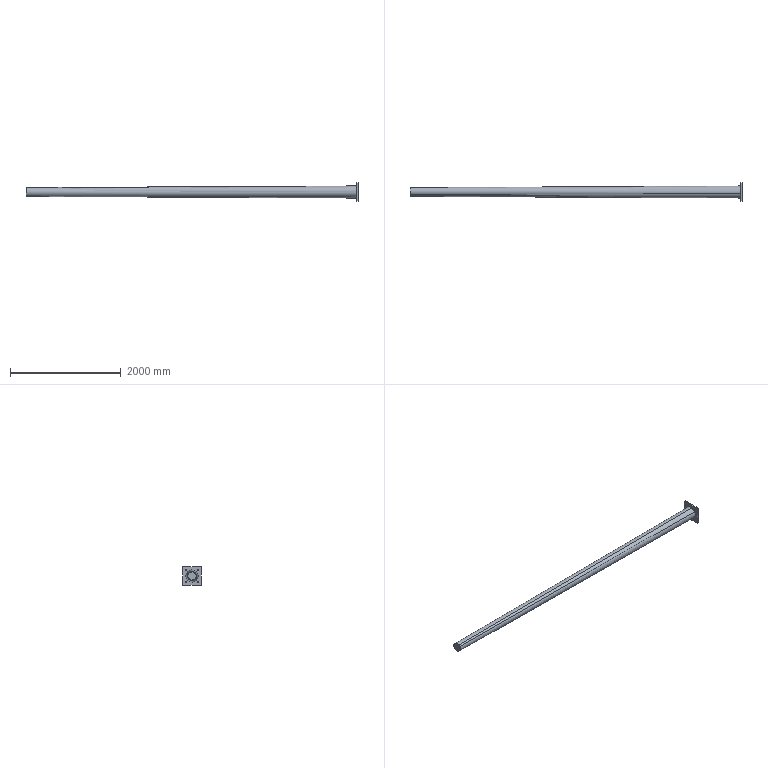Component | SolidWorks | Cantilever-1 | 1 solid | 20 faces | box 6000 x 330 x 330 mm | volume 23316974 mm3 | cylinder 8 | plane 8 | spline 2 | cone 2 | commonest cylinder face diameters 16 x8
STEP:
#1=COLOUR_RGB('',0.7922,0.8196,0.9333);
#2=FILL_AREA_STYLE_COLOUR('',#1);
#3=FILL_AREA_STYLE('',(#2));
#4=SURFACE_STYLE_FILL_AREA(#3);
#5=SURFACE_SIDE_STYLE('',(#4));
#6=SURFACE_STYLE_USAGE(.BOTH.,#5);
#7=PRESENTATION_STYLE_ASSIGNMENT((#6));
#8=CARTESIAN_POINT('',(-8.524,280.032,-4.345));
#9=VERTEX_POINT('',#8);
#10=CARTESIAN_POINT('',(-8.524,279.501,-4.007));
#11=VERTEX_POINT('',#10);
#12=CARTESIAN_POINT('',(-8.524,279.766,-4.176));
#13=DIRECTION('',(-1.,-0.,-0.));
#14=DIRECTION('',(0.,0.5373,0.8434));
#15=AXIS2_PLACEMENT_3D('',#12,#13,#14);
#16=CIRCLE('',#15,0.315);
#17=EDGE_CURVE('',#9,#11,#16,.T.);
#18=ORIENTED_EDGE('',*,*,#17,.F.);
#19=CARTESIAN_POINT('',(-9.311,280.032,-4.345));
#20=VERTEX_POINT('',#19);
#21=CARTESIAN_POINT('',(-8.524,280.032,-4.345));
#22=DIRECTION('',(-1.,-0.,-0.));
#23=VECTOR('',#22,39.37);
#24=LINE('',#21,#23);
#25=EDGE_CURVE('',#9,#20,#24,.T.);
#26=ORIENTED_EDGE('',*,*,#25,.T.);
#27=CARTESIAN_POINT('',(-9.311,279.501,-4.007));
#28=VERTEX_POINT('',#27);
#29=CARTESIAN_POINT('',(-9.311,279.766,-4.176));
#30=DIRECTION('',(-1.,-0.,-0.));
#31=DIRECTION('',(0.,0.5373,0.8434));
#32=AXIS2_PLACEMENT_3D('',#29,#30,#31);
#33=CIRCLE('',#32,0.315);
#34=EDGE_CURVE('',#20,#28,#33,.T.);
#35=ORIENTED_EDGE('',*,*,#34,.T.);
#36=CARTESIAN_POINT('',(-8.524,279.501,-4.007));
#37=DIRECTION('',(-1.,-0.,-0.));
#38=VECTOR('',#37,39.37);
#39=LINE('',#36,#38);
#40=EDGE_CURVE('',#11,#28,#39,.T.);
#41=ORIENTED_EDGE('',*,*,#40,.F.);
#42=EDGE_LOOP('',(#18,#26,#35,#41));
#43=FACE_OUTER_BOUND('',#42,.T.);
#44=CARTESIAN_POINT('',(-8.524,279.766,-4.176));
#45=DIRECTION('',(-1.,-0.,-0.));
#46=DIRECTION('',(0.,-0.8434,0.5373));
#47=AXIS2_PLACEMENT_3D('',#44,#45,#46);
#48=CYLINDRICAL_SURFACE('',#47,0.315);
#49=ADVANCED_FACE('',(#43),#48,.F.);
#50=CARTESIAN_POINT('',(-8.524,271.68,-4.345));
#51=VERTEX_POINT('',#50);
#52=CARTESIAN_POINT('',(-8.524,271.149,-4.007));
#53=VERTEX_POINT('',#52);
#54=CARTESIAN_POINT('',(-8.524,271.415,-4.176));
#55=DIRECTION('',(-1.,-0.,-0.));
#56=DIRECTION('',(0.,0.8434,-0.5373));
#57=AXIS2_PLACEMENT_3D('',#54,#55,#56);
#58=CIRCLE('',#57,0.315);
#59=EDGE_CURVE('',#51,#53,#58,.T.);
#60=ORIENTED_EDGE('',*,*,#59,.F.);
#61=CARTESIAN_POINT('',(-9.311,271.68,-4.345));
#62=VERTEX_POINT('',#61);
#63=CARTESIAN_POINT('',(-8.524,271.68,-4.345));
#64=DIRECTION('',(-1.,-0.,-0.));
#65=VECTOR('',#64,39.37);
#66=LINE('',#63,#65);
#67=EDGE_CURVE('',#51,#62,#66,.T.);
#68=ORIENTED_EDGE('',*,*,#67,.T.);
#69=CARTESIAN_POINT('',(-9.311,271.149,-4.007));
#70=VERTEX_POINT('',#69);
#71=CARTESIAN_POINT('',(-9.311,271.415,-4.176));
#72=DIRECTION('',(-1.,-0.,-0.));
#73=DIRECTION('',(0.,0.8434,-0.5373));
#74=AXIS2_PLACEMENT_3D('',#71,#72,#73);
#75=CIRCLE('',#74,0.315);
#76=EDGE_CURVE('',#62,#70,#75,.T.);
#77=ORIENTED_EDGE('',*,*,#76,.T.);
#78=CARTESIAN_POINT('',(-8.524,271.149,-4.007));
#79=DIRECTION('',(-1.,-0.,-0.));
#80=VECTOR('',#79,39.37);
#81=LINE('',#78,#80);
#82=EDGE_CURVE('',#53,#70,#81,.T.);
#83=ORIENTED_EDGE('',*,*,#82,.F.);
#84=EDGE_LOOP('',(#60,#68,#77,#83));
#85=FACE_OUTER_BOUND('',#84,.T.);
#86=CARTESIAN_POINT('',(-8.524,271.415,-4.176));
#87=DIRECTION('',(-1.,-0.,-0.));
#88=DIRECTION('',(0.,-0.8434,0.5373));
#89=AXIS2_PLACEMENT_3D('',#86,#87,#88);
#90=CYLINDRICAL_SURFACE('',#89,0.315);
#91=ADVANCED_FACE('',(#85),#90,.F.);
#92=CARTESIAN_POINT('',(-8.524,271.68,4.007));
#93=VERTEX_POINT('',#92);
#94=CARTESIAN_POINT('',(-8.524,271.149,4.345));
#95=VERTEX_POINT('',#94);
#96=CARTESIAN_POINT('',(-8.524,271.415,4.176));
#97=DIRECTION('',(-1.,-0.,-0.));
#98=DIRECTION('',(0.,-0.5373,-0.8434));
#99=AXIS2_PLACEMENT_3D('',#96,#97,#98);
#100=CIRCLE('',#99,0.315);
#101=EDGE_CURVE('',#93,#95,#100,.T.);
#102=ORIENTED_EDGE('',*,*,#101,.F.);
#103=CARTESIAN_POINT('',(-9.311,271.68,4.007));
#104=VERTEX_POINT('',#103);
#105=CARTESIAN_POINT('',(-8.524,271.68,4.007));
#106=DIRECTION('',(-1.,-0.,-0.));
#107=VECTOR('',#106,39.37);
#108=LINE('',#105,#107);
#109=EDGE_CURVE('',#93,#104,#108,.T.);
#110=ORIENTED_EDGE('',*,*,#109,.T.);
#111=CARTESIAN_POINT('',(-9.311,271.149,4.345));
#112=VERTEX_POINT('',#111);
#113=CARTESIAN_POINT('',(-9.311,271.415,4.176));
#114=DIRECTION('',(-1.,-0.,-0.));
#115=DIRECTION('',(0.,-0.5373,-0.8434));
#116=AXIS2_PLACEMENT_3D('',#113,#114,#115);
#117=CIRCLE('',#116,0.315);
#118=EDGE_CURVE('',#104,#112,#117,.T.);
#119=ORIENTED_EDGE('',*,*,#118,.T.);
#120=CARTESIAN_POINT('',(-8.524,271.149,4.345));
#121=DIRECTION('',(-1.,-0.,-0.));
#122=VECTOR('',#121,39.37);
#123=LINE('',#120,#122);
#124=EDGE_CURVE('',#95,#112,#123,.T.);
#125=ORIENTED_EDGE('',*,*,#124,.F.);
#126=EDGE_LOOP('',(#102,#110,#119,#125));
#127=FACE_OUTER_BOUND('',#126,.T.);
#128=CARTESIAN_POINT('',(-8.524,271.415,4.176));
#129=DIRECTION('',(-1.,-0.,-0.));
#130=DIRECTION('',(0.,-0.8434,0.5373));
#131=AXIS2_PLACEMENT_3D('',#128,#129,#130);
#132=CYLINDRICAL_SURFACE('',#131,0.315);
#133=ADVANCED_FACE('',(#127),#132,.F.);
#134=CARTESIAN_POINT('',(-8.524,280.032,4.007));
#135=VERTEX_POINT('',#134);
#136=CARTESIAN_POINT('',(-8.524,279.501,4.345));
#137=VERTEX_POINT('',#136);
#138=CARTESIAN_POINT('',(-8.524,279.766,4.176));
#139=DIRECTION('',(-1.,-0.,-0.));
#140=DIRECTION('',(0.,-0.8434,0.5373));
#141=AXIS2_PLACEMENT_3D('',#138,#139,#140);
#142=CIRCLE('',#141,0.315);
#143=EDGE_CURVE('',#135,#137,#142,.T.);
#144=ORIENTED_EDGE('',*,*,#143,.F.);
#145=CARTESIAN_POINT('',(-9.311,280.032,4.007));
#146=VERTEX_POINT('',#145);
#147=CARTESIAN_POINT('',(-8.524,280.032,4.007));
#148=DIRECTION('',(-1.,-0.,-0.));
#149=VECTOR('',#148,39.37);
#150=LINE('',#147,#149);
#151=EDGE_CURVE('',#135,#146,#150,.T.);
#152=ORIENTED_EDGE('',*,*,#151,.T.);
#153=CARTESIAN_POINT('',(-9.311,279.501,4.345));
#154=VERTEX_POINT('',#153);
#155=CARTESIAN_POINT('',(-9.311,279.766,4.176));
#156=DIRECTION('',(-1.,-0.,-0.));
#157=DIRECTION('',(0.,-0.8434,0.5373));
#158=AXIS2_PLACEMENT_3D('',#155,#156,#157);
#159=CIRCLE('',#158,0.315);
#160=EDGE_CURVE('',#146,#154,#159,.T.);
#161=ORIENTED_EDGE('',*,*,#160,.T.);
#162=CARTESIAN_POINT('',(-8.524,279.501,4.345));
#163=DIRECTION('',(-1.,-0.,-0.));
#164=VECTOR('',#163,39.37);
#165=LINE('',#162,#164);
#166=EDGE_CURVE('',#137,#154,#165,.T.);
#167=ORIENTED_EDGE('',*,*,#166,.F.);
#168=EDGE_LOOP('',(#144,#152,#161,#167));
#169=FACE_OUTER_BOUND('',#168,.T.);
#170=CARTESIAN_POINT('',(-8.524,279.766,4.176));
#171=DIRECTION('',(-1.,-0.,-0.));
#172=DIRECTION('',(0.,-0.8434,0.5373));
#173=AXIS2_PLACEMENT_3D('',#170,#171,#172);
#174=CYLINDRICAL_SURFACE('',#173,0.315);
#175=ADVANCED_FACE('',(#169),#174,.F.);
#176=CARTESIAN_POINT('',(-244.744,277.198,-2.686));
#177=VERTEX_POINT('',#176);
#178=CARTESIAN_POINT('',(-244.744,273.983,2.686));
#179=VERTEX_POINT('',#178);
#180=CARTESIAN_POINT('',(-244.744,275.591,0.));
#181=DIRECTION('',(-1.,-0.,-0.));
#182=DIRECTION('',(0.,-0.8434,0.5373));
#183=AXIS2_PLACEMENT_3D('',#180,#181,#182);
#184=CIRCLE('',#183,3.13);
#185=EDGE_CURVE('',#177,#179,#184,.T.);
#186=ORIENTED_EDGE('',*,*,#185,.F.);
#187=CARTESIAN_POINT('',(-9.311,276.61,-4.184));
#188=VERTEX_POINT('',#187);
#189=CARTESIAN_POINT('',(-244.744,277.198,-2.686));
#190=CARTESIAN_POINT('',(-9.311,276.61,-4.184));
#191=B_SPLINE_CURVE_WITH_KNOTS('',1,(#189,#190),.UNSPECIFIED.,.F.,.F.,(2,2),(0.,0.9967),.UNSPECIFIED.);
#192=EDGE_CURVE('',#177,#188,#191,.T.);
#193=ORIENTED_EDGE('',*,*,#192,.T.);
#194=CARTESIAN_POINT('',(-9.311,274.571,4.184));
#195=VERTEX_POINT('',#194);
#196=CARTESIAN_POINT('',(-9.311,275.591,0.));
#197=DIRECTION('',(-1.,-0.,-0.));
#198=DIRECTION('',(0.,0.8434,-0.5373));
#199=AXIS2_PLACEMENT_3D('',#196,#197,#198);
#200=CIRCLE('',#199,4.307);
#201=EDGE_CURVE('',#188,#195,#200,.T.);
#202=ORIENTED_EDGE('',*,*,#201,.T.);
#203=CARTESIAN_POINT('',(-244.744,273.983,2.686));
#204=CARTESIAN_POINT('',(-9.311,274.571,4.184));
#205=B_SPLINE_CURVE_WITH_KNOTS('',1,(#203,#204),.UNSPECIFIED.,.F.,.F.,(2,2),(0.,0.9967),.UNSPECIFIED.);
#206=EDGE_CURVE('',#179,#195,#205,.T.);
#207=ORIENTED_EDGE('',*,*,#206,.F.);
#208=EDGE_LOOP('',(#186,#193,#202,#207));
#209=FACE_OUTER_BOUND('',#208,.T.);
#210=CARTESIAN_POINT('',(-244.744,273.983,2.686));
#211=CARTESIAN_POINT('',(-8.524,274.573,4.189));
#212=CARTESIAN_POINT('',(-244.744,268.612,-0.5283));
#213=CARTESIAN_POINT('',(-8.524,266.195,2.155));
#214=CARTESIAN_POINT('',(-244.744,271.826,-5.9));
#215=CARTESIAN_POINT('',(-8.524,268.229,-6.224));
#216=CARTESIAN_POINT('',(-244.744,277.198,-2.686));
#217=CARTESIAN_POINT('',(-8.524,276.608,-4.189));
#218=CARTESIAN_POINT('',(-244.744,282.569,0.5283));
#219=CARTESIAN_POINT('',(-8.524,284.986,-2.155));
#220=CARTESIAN_POINT('',(-244.744,279.355,5.9));
#221=CARTESIAN_POINT('',(-8.524,282.952,6.224));
#222=CARTESIAN_POINT('',(-244.744,273.983,2.686));
#223=CARTESIAN_POINT('',(-8.524,274.573,4.189));
#224=(BOUNDED_SURFACE()B_SPLINE_SURFACE(3,1,((#210,#211),(#212,#213),(#214,#215),(#216,#217),(#218,#219),(#220,#221),(#222,#223)),.UNSPECIFIED.,.T.,.F.,.T.)B_SPLINE_SURFACE_WITH_KNOTS((4,3,4),(2,2),(0.,0.5,1.),(0.,1.),.UNSPECIFIED.)GEOMETRIC_REPRESENTATION_ITEM()RATIONAL_B_SPLINE_SURFACE(((1.,1.),(0.3333,0.3333),(0.3333,0.3333),(1.,1.),(0.3333,0.3333),(0.3333,0.3333),(1.,1.)))REPRESENTATION_ITEM('')SURFACE());
#225=ADVANCED_FACE('',(#209),#224,.T.);
#226=CARTESIAN_POINT('',(-244.35,273.149,1.556));
#227=VERTEX_POINT('',#226);
#228=CARTESIAN_POINT('',(-244.35,278.033,-1.556));
#229=VERTEX_POINT('',#228);
#230=CARTESIAN_POINT('',(-244.35,275.591,0.));
#231=DIRECTION('',(1.,0.,0.));
#232=DIRECTION('',(0.,-0.8434,0.5373));
#233=AXIS2_PLACEMENT_3D('',#230,#231,#232);
#234=CIRCLE('',#233,2.896);
#235=EDGE_CURVE('',#227,#229,#234,.T.);
#236=ORIENTED_EDGE('',*,*,#235,.F.);
#237=CARTESIAN_POINT('',(-8.524,272.22,2.147));
#238=VERTEX_POINT('',#237);
#239=CARTESIAN_POINT('',(-244.744,273.15,1.555));
#240=DIRECTION('',(1.,-0.003936,0.002507));
#241=VECTOR('',#240,39.37);
#242=LINE('',#239,#241);
#243=EDGE_CURVE('',#227,#238,#242,.T.);
#244=ORIENTED_EDGE('',*,*,#243,.T.);
#245=CARTESIAN_POINT('',(-8.524,278.961,-2.147));
#246=VERTEX_POINT('',#245);
#247=CARTESIAN_POINT('',(-8.524,275.591,0.));
#248=DIRECTION('',(-1.,-0.,-0.));
#249=DIRECTION('',(0.,-0.8434,0.5373));
#250=AXIS2_PLACEMENT_3D('',#247,#248,#249);
#251=CIRCLE('',#250,3.996);
#252=EDGE_CURVE('',#246,#238,#251,.T.);
#253=ORIENTED_EDGE('',*,*,#252,.F.);
#254=CARTESIAN_POINT('',(-244.744,278.031,-1.555));
#255=DIRECTION('',(1.,0.003936,-0.002507));
#256=VECTOR('',#255,39.37);
#257=LINE('',#254,#256);
#258=EDGE_CURVE('',#229,#246,#257,.T.);
#259=ORIENTED_EDGE('',*,*,#258,.F.);
#260=EDGE_LOOP('',(#236,#244,#253,#259));
#261=FACE_OUTER_BOUND('',#260,.T.);
#262=CARTESIAN_POINT('',(-244.744,275.591,0.));
#263=DIRECTION('',(1.,0.,0.));
#264=DIRECTION('',(0.,0.8434,-0.5373));
#265=AXIS2_PLACEMENT_3D('',#262,#263,#264);
#266=CONICAL_SURFACE('',#265,2.894,0.004667);
#267=ADVANCED_FACE('',(#261),#266,.F.);
#268=ORIENTED_EDGE('',*,*,#243,.F.);
#269=CARTESIAN_POINT('',(-244.35,275.591,0.));
#270=DIRECTION('',(1.,0.,0.));
#271=DIRECTION('',(0.,-0.8434,0.5373));
#272=AXIS2_PLACEMENT_3D('',#269,#270,#271);
#273=CIRCLE('',#272,2.896);
#274=EDGE_CURVE('',#229,#227,#273,.T.);
#275=ORIENTED_EDGE('',*,*,#274,.F.);
#276=ORIENTED_EDGE('',*,*,#258,.T.);
#277=CARTESIAN_POINT('',(-8.524,275.591,0.));
#278=DIRECTION('',(-1.,-0.,-0.));
#279=DIRECTION('',(0.,-0.8434,0.5373));
#280=AXIS2_PLACEMENT_3D('',#277,#278,#279);
#281=CIRCLE('',#280,3.996);
#282=EDGE_CURVE('',#238,#246,#281,.T.);
#283=ORIENTED_EDGE('',*,*,#282,.F.);
#284=EDGE_LOOP('',(#268,#275,#276,#283));
#285=FACE_OUTER_BOUND('',#284,.T.);
#286=CARTESIAN_POINT('',(-244.744,275.591,0.));
#287=DIRECTION('',(1.,0.,0.));
#288=DIRECTION('',(0.,0.8434,-0.5373));
#289=AXIS2_PLACEMENT_3D('',#286,#287,#288);
#290=CONICAL_SURFACE('',#289,2.894,0.004667);
#291=ADVANCED_FACE('',(#285),#290,.F.);
#292=ORIENTED_EDGE('',*,*,#192,.F.);
#293=CARTESIAN_POINT('',(-244.744,275.591,0.));
#294=DIRECTION('',(-1.,-0.,-0.));
#295=DIRECTION('',(0.,-0.8434,0.5373));
#296=AXIS2_PLACEMENT_3D('',#293,#294,#295);
#297=CIRCLE('',#296,3.13);
#298=EDGE_CURVE('',#179,#177,#297,.T.);
#299=ORIENTED_EDGE('',*,*,#298,.F.);
#300=ORIENTED_EDGE('',*,*,#206,.T.);
#301=CARTESIAN_POINT('',(-9.311,275.591,0.));
#302=DIRECTION('',(-1.,-0.,-0.));
#303=DIRECTION('',(0.,0.8434,-0.5373));
#304=AXIS2_PLACEMENT_3D('',#301,#302,#303);
#305=CIRCLE('',#304,4.307);
#306=EDGE_CURVE('',#195,#188,#305,.T.);
#307=ORIENTED_EDGE('',*,*,#306,.T.);
#308=EDGE_LOOP('',(#292,#299,#300,#307));
#309=FACE_OUTER_BOUND('',#308,.T.);
#310=CARTESIAN_POINT('',(-244.744,273.983,2.686));
#311=CARTESIAN_POINT('',(-8.524,274.573,4.189));
#312=CARTESIAN_POINT('',(-244.744,268.612,-0.5283));
#313=CARTESIAN_POINT('',(-8.524,266.195,2.155));
#314=CARTESIAN_POINT('',(-244.744,271.826,-5.9));
#315=CARTESIAN_POINT('',(-8.524,268.229,-6.224));
#316=CARTESIAN_POINT('',(-244.744,277.198,-2.686));
#317=CARTESIAN_POINT('',(-8.524,276.608,-4.189));
#318=CARTESIAN_POINT('',(-244.744,282.569,0.5283));
#319=CARTESIAN_POINT('',(-8.524,284.986,-2.155));
#320=CARTESIAN_POINT('',(-244.744,279.355,5.9));
#321=CARTESIAN_POINT('',(-8.524,282.952,6.224));
#322=CARTESIAN_POINT('',(-244.744,273.983,2.686));
#323=CARTESIAN_POINT('',(-8.524,274.573,4.189));
#324=(BOUNDED_SURFACE()B_SPLINE_SURFACE(3,1,((#310,#311),(#312,#313),(#314,#315),(#316,#317),(#318,#319),(#320,#321),(#322,#323)),.UNSPECIFIED.,.T.,.F.,.F.)B_SPLINE_SURFACE_WITH_KNOTS((4,3,4),(2,2),(0.,0.5,1.),(0.,1.),.UNSPECIFIED.)GEOMETRIC_REPRESENTATION_ITEM()RATIONAL_B_SPLINE_SURFACE(((1.,1.),(0.3333,0.3333),(0.3333,0.3333),(1.,1.),(0.3333,0.3333),(0.3333,0.3333),(1.,1.)))REPRESENTATION_ITEM('')SURFACE());
#325=ADVANCED_FACE('',(#309),#324,.T.);
#326=CARTESIAN_POINT('',(-8.524,279.766,-4.176));
#327=DIRECTION('',(-1.,-0.,-0.));
#328=DIRECTION('',(0.,0.5373,0.8434));
#329=AXIS2_PLACEMENT_3D('',#326,#327,#328);
#330=CIRCLE('',#329,0.315);
#331=EDGE_CURVE('',#11,#9,#330,.T.);
#332=ORIENTED_EDGE('',*,*,#331,.T.);
#333=ORIENTED_EDGE('',*,*,#17,.T.);
#334=EDGE_LOOP('',(#332,#333));
#335=FACE_BOUND('',#334,.T.);
#336=CARTESIAN_POINT('',(-8.524,271.415,-4.176));
#337=DIRECTION('',(-1.,-0.,-0.));
#338=DIRECTION('',(0.,0.8434,-0.5373));
#339=AXIS2_PLACEMENT_3D('',#336,#337,#338);
#340=CIRCLE('',#339,0.315);
#341=EDGE_CURVE('',#53,#51,#340,.T.);
#342=ORIENTED_EDGE('',*,*,#341,.T.);
#343=ORIENTED_EDGE('',*,*,#59,.T.);
#344=EDGE_LOOP('',(#342,#343));
#345=FACE_BOUND('',#344,.T.);
#346=CARTESIAN_POINT('',(-8.524,271.415,4.176));
#347=DIRECTION('',(-1.,-0.,-0.));
#348=DIRECTION('',(0.,-0.5373,-0.8434));
#349=AXIS2_PLACEMENT_3D('',#346,#347,#348);
#350=CIRCLE('',#349,0.315);
#351=EDGE_CURVE('',#95,#93,#350,.T.);
#352=ORIENTED_EDGE('',*,*,#351,.T.);
#353=ORIENTED_EDGE('',*,*,#101,.T.);
#354=EDGE_LOOP('',(#352,#353));
#355=FACE_BOUND('',#354,.T.);
#356=CARTESIAN_POINT('',(-8.524,279.766,4.176));
#357=DIRECTION('',(-1.,-0.,-0.));
#358=DIRECTION('',(0.,-0.8434,0.5373));
#359=AXIS2_PLACEMENT_3D('',#356,#357,#358);
#360=CIRCLE('',#359,0.315);
#361=EDGE_CURVE('',#137,#135,#360,.T.);
#362=ORIENTED_EDGE('',*,*,#361,.T.);
#363=ORIENTED_EDGE('',*,*,#143,.T.);
#364=EDGE_LOOP('',(#362,#363));
#365=FACE_BOUND('',#364,.T.);
#366=ORIENTED_EDGE('',*,*,#252,.T.);
#367=ORIENTED_EDGE('',*,*,#282,.T.);
#368=EDGE_LOOP('',(#366,#367));
#369=FACE_BOUND('',#368,.T.);
#370=CARTESIAN_POINT('',(-8.524,269.094,-6.496));
#371=VERTEX_POINT('',#370);
#372=CARTESIAN_POINT('',(-8.524,282.087,-6.496));
#373=VERTEX_POINT('',#372);
#374=CARTESIAN_POINT('',(-8.524,269.094,-6.496));
#375=DIRECTION('',(-0.,1.,0.));
#376=VECTOR('',#375,39.37);
#377=LINE('',#374,#376);
#378=EDGE_CURVE('',#371,#373,#377,.T.);
#379=ORIENTED_EDGE('',*,*,#378,.T.);
#380=CARTESIAN_POINT('',(-8.524,282.087,6.496));
#381=VERTEX_POINT('',#380);
#382=CARTESIAN_POINT('',(-8.524,282.087,-6.496));
#383=DIRECTION('',(-0.,-0.,1.));
#384=VECTOR('',#383,39.37);
#385=LINE('',#382,#384);
#386=EDGE_CURVE('',#373,#381,#385,.T.);
#387=ORIENTED_EDGE('',*,*,#386,.T.);
#388=CARTESIAN_POINT('',(-8.524,269.094,6.496));
#389=VERTEX_POINT('',#388);
#390=CARTESIAN_POINT('',(-8.524,282.087,6.496));
#391=DIRECTION('',(0.,-1.,0.));
#392=VECTOR('',#391,39.37);
#393=LINE('',#390,#392);
#394=EDGE_CURVE('',#381,#389,#393,.T.);
#395=ORIENTED_EDGE('',*,*,#394,.T.);
#396=CARTESIAN_POINT('',(-8.524,269.094,6.496));
#397=DIRECTION('',(0.,0.,-1.));
#398=VECTOR('',#397,39.37);
#399=LINE('',#396,#398);
#400=EDGE_CURVE('',#389,#371,#399,.T.);
#401=ORIENTED_EDGE('',*,*,#400,.T.);
#402=EDGE_LOOP('',(#379,#387,#395,#401));
#403=FACE_OUTER_BOUND('',#402,.T.);
#404=CARTESIAN_POINT('',(-8.524,275.591,0.));
#405=DIRECTION('',(-1.,-0.,-0.));
#406=DIRECTION('',(0.,-0.8434,0.5373));
#407=AXIS2_PLACEMENT_3D('',#404,#405,#406);
#408=PLANE('',#407);
#409=ADVANCED_FACE('',(#335,#345,#355,#365,#369,#403),#408,.F.);
#410=ORIENTED_EDGE('',*,*,#298,.T.);
#411=ORIENTED_EDGE('',*,*,#185,.T.);
#412=EDGE_LOOP('',(#410,#411));
#413=FACE_OUTER_BOUND('',#412,.T.);
#414=CARTESIAN_POINT('',(-244.744,275.591,0.));
#415=DIRECTION('',(-1.,-0.,-0.));
#416=DIRECTION('',(0.,-0.8434,0.5373));
#417=AXIS2_PLACEMENT_3D('',#414,#415,#416);
#418=PLANE('',#417);
#419=ADVANCED_FACE('',(#413),#418,.T.);
#420=ORIENTED_EDGE('',*,*,#378,.F.);
#421=CARTESIAN_POINT('',(-9.311,269.094,-6.496));
#422=VERTEX_POINT('',#421);
#423=CARTESIAN_POINT('',(-9.311,269.094,-6.496));
#424=DIRECTION('',(1.,0.,0.));
#425=VECTOR('',#424,39.37);
#426=LINE('',#423,#425);
#427=EDGE_CURVE('',#422,#371,#426,.T.);
#428=ORIENTED_EDGE('',*,*,#427,.F.);
#429=CARTESIAN_POINT('',(-9.311,282.087,-6.496));
#430=VERTEX_POINT('',#429);
#431=CARTESIAN_POINT('',(-9.311,269.094,-6.496));
#432=DIRECTION('',(-0.,1.,0.));
#433=VECTOR('',#432,39.37);
#434=LINE('',#431,#433);
#435=EDGE_CURVE('',#422,#430,#434,.T.);
#436=ORIENTED_EDGE('',*,*,#435,.T.);
#437=CARTESIAN_POINT('',(-9.311,282.087,-6.496));
#438=DIRECTION('',(1.,0.,0.));
#439=VECTOR('',#438,39.37);
#440=LINE('',#437,#439);
#441=EDGE_CURVE('',#430,#373,#440,.T.);
#442=ORIENTED_EDGE('',*,*,#441,.T.);
#443=EDGE_LOOP('',(#420,#428,#436,#442));
#444=FACE_OUTER_BOUND('',#443,.T.);
#445=CARTESIAN_POINT('',(-9.311,269.094,-6.496));
#446=DIRECTION('',(0.,0.,-1.));
#447=DIRECTION('',(0.,-1.,-0.));
#448=AXIS2_PLACEMENT_3D('',#445,#446,#447);
#449=PLANE('',#448);
#450=ADVANCED_FACE('',(#444),#449,.T.);
#451=ORIENTED_EDGE('',*,*,#400,.F.);
#452=CARTESIAN_POINT('',(-9.311,269.094,6.496));
#453=VERTEX_POINT('',#452);
#454=CARTESIAN_POINT('',(-9.311,269.094,6.496));
#455=DIRECTION('',(1.,0.,0.));
#456=VECTOR('',#455,39.37);
#457=LINE('',#454,#456);
#458=EDGE_CURVE('',#453,#389,#457,.T.);
#459=ORIENTED_EDGE('',*,*,#458,.F.);
#460=CARTESIAN_POINT('',(-9.311,269.094,6.496));
#461=DIRECTION('',(0.,0.,-1.));
#462=VECTOR('',#461,39.37);
#463=LINE('',#460,#462);
#464=EDGE_CURVE('',#453,#422,#463,.T.);
#465=ORIENTED_EDGE('',*,*,#464,.T.);
#466=ORIENTED_EDGE('',*,*,#427,.T.);
#467=EDGE_LOOP('',(#451,#459,#465,#466));
#468=FACE_OUTER_BOUND('',#467,.T.);
#469=CARTESIAN_POINT('',(-9.311,269.094,6.496));
#470=DIRECTION('',(0.,-1.,-0.));
#471=DIRECTION('',(-0.,-0.,1.));
#472=AXIS2_PLACEMENT_3D('',#469,#470,#471);
#473=PLANE('',#472);
#474=ADVANCED_FACE('',(#468),#473,.T.);
#475=ORIENTED_EDGE('',*,*,#394,.F.);
#476=CARTESIAN_POINT('',(-9.311,282.087,6.496));
#477=VERTEX_POINT('',#476);
#478=CARTESIAN_POINT('',(-9.311,282.087,6.496));
#479=DIRECTION('',(1.,0.,0.));
#480=VECTOR('',#479,39.37);
#481=LINE('',#478,#480);
#482=EDGE_CURVE('',#477,#381,#481,.T.);
#483=ORIENTED_EDGE('',*,*,#482,.F.);
#484=CARTESIAN_POINT('',(-9.311,282.087,6.496));
#485=DIRECTION('',(0.,-1.,0.));
#486=VECTOR('',#485,39.37);
#487=LINE('',#484,#486);
#488=EDGE_CURVE('',#477,#453,#487,.T.);
#489=ORIENTED_EDGE('',*,*,#488,.T.);
#490=ORIENTED_EDGE('',*,*,#458,.T.);
#491=EDGE_LOOP('',(#475,#483,#489,#490));
#492=FACE_OUTER_BOUND('',#491,.T.);
#493=CARTESIAN_POINT('',(-9.311,282.087,6.496));
#494=DIRECTION('',(-0.,0.,1.));
#495=DIRECTION('',(-0.,1.,-0.));
#496=AXIS2_PLACEMENT_3D('',#493,#494,#495);
#497=PLANE('',#496);
#498=ADVANCED_FACE('',(#492),#497,.T.);
#499=ORIENTED_EDGE('',*,*,#386,.F.);
#500=ORIENTED_EDGE('',*,*,#441,.F.);
#501=CARTESIAN_POINT('',(-9.311,282.087,-6.496));
#502=DIRECTION('',(-0.,-0.,1.));
#503=VECTOR('',#502,39.37);
#504=LINE('',#501,#503);
#505=EDGE_CURVE('',#430,#477,#504,.T.);
#506=ORIENTED_EDGE('',*,*,#505,.T.);
#507=ORIENTED_EDGE('',*,*,#482,.T.);
#508=EDGE_LOOP('',(#499,#500,#506,#507));
#509=FACE_OUTER_BOUND('',#508,.T.);
#510=CARTESIAN_POINT('',(-9.311,282.087,-6.496));
#511=DIRECTION('',(-0.,1.,0.));
#512=DIRECTION('',(0.,0.,-1.));
#513=AXIS2_PLACEMENT_3D('',#510,#511,#512);
#514=PLANE('',#513);
#515=ADVANCED_FACE('',(#509),#514,.T.);
#516=CARTESIAN_POINT('',(-9.311,279.766,-4.176));
#517=DIRECTION('',(-1.,-0.,-0.));
#518=DIRECTION('',(0.,0.5373,0.8434));
#519=AXIS2_PLACEMENT_3D('',#516,#517,#518);
#520=CIRCLE('',#519,0.315);
#521=EDGE_CURVE('',#28,#20,#520,.T.);
#522=ORIENTED_EDGE('',*,*,#521,.F.);
#523=ORIENTED_EDGE('',*,*,#34,.F.);
#524=EDGE_LOOP('',(#522,#523));
#525=FACE_BOUND('',#524,.T.);
#526=CARTESIAN_POINT('',(-9.311,271.415,-4.176));
#527=DIRECTION('',(-1.,-0.,-0.));
#528=DIRECTION('',(0.,0.8434,-0.5373));
#529=AXIS2_PLACEMENT_3D('',#526,#527,#528);
#530=CIRCLE('',#529,0.315);
#531=EDGE_CURVE('',#70,#62,#530,.T.);
#532=ORIENTED_EDGE('',*,*,#531,.F.);
#533=ORIENTED_EDGE('',*,*,#76,.F.);
#534=EDGE_LOOP('',(#532,#533));
#535=FACE_BOUND('',#534,.T.);
#536=CARTESIAN_POINT('',(-9.311,271.415,4.176));
#537=DIRECTION('',(-1.,-0.,-0.));
#538=DIRECTION('',(0.,-0.5373,-0.8434));
#539=AXIS2_PLACEMENT_3D('',#536,#537,#538);
#540=CIRCLE('',#539,0.315);
#541=EDGE_CURVE('',#112,#104,#540,.T.);
#542=ORIENTED_EDGE('',*,*,#541,.F.);
#543=ORIENTED_EDGE('',*,*,#118,.F.);
#544=EDGE_LOOP('',(#542,#543));
#545=FACE_BOUND('',#544,.T.);
#546=CARTESIAN_POINT('',(-9.311,279.766,4.176));
#547=DIRECTION('',(-1.,-0.,-0.));
#548=DIRECTION('',(0.,-0.8434,0.5373));
#549=AXIS2_PLACEMENT_3D('',#546,#547,#548);
#550=CIRCLE('',#549,0.315);
#551=EDGE_CURVE('',#154,#146,#550,.T.);
#552=ORIENTED_EDGE('',*,*,#551,.F.);
#553=ORIENTED_EDGE('',*,*,#160,.F.);
#554=EDGE_LOOP('',(#552,#553));
#555=FACE_BOUND('',#554,.T.);
#556=ORIENTED_EDGE('',*,*,#306,.F.);
#557=ORIENTED_EDGE('',*,*,#201,.F.);
#558=EDGE_LOOP('',(#556,#557));
#559=FACE_BOUND('',#558,.T.);
#560=ORIENTED_EDGE('',*,*,#435,.F.);
#561=ORIENTED_EDGE('',*,*,#464,.F.);
#562=ORIENTED_EDGE('',*,*,#488,.F.);
#563=ORIENTED_EDGE('',*,*,#505,.F.);
#564=EDGE_LOOP('',(#560,#561,#562,#563));
#565=FACE_OUTER_BOUND('',#564,.T.);
#566=CARTESIAN_POINT('',(-9.311,108.152,-262.807));
#567=DIRECTION('',(1.,0.,0.));
#568=DIRECTION('',(-0.,0.8434,-0.5373));
#569=AXIS2_PLACEMENT_3D('',#566,#567,#568);
#570=PLANE('',#569);
#571=ADVANCED_FACE('',(#525,#535,#545,#555,#559,#565),#570,.F.);
#572=ORIENTED_EDGE('',*,*,#151,.F.);
#573=ORIENTED_EDGE('',*,*,#361,.F.);
#574=ORIENTED_EDGE('',*,*,#166,.T.);
#575=ORIENTED_EDGE('',*,*,#551,.T.);
#576=EDGE_LOOP('',(#572,#573,#574,#575));
#577=FACE_OUTER_BOUND('',#576,.T.);
#578=CARTESIAN_POINT('',(-8.524,279.766,4.176));
#579=DIRECTION('',(-1.,-0.,-0.));
#580=DIRECTION('',(0.,-0.8434,0.5373));
#581=AXIS2_PLACEMENT_3D('',#578,#579,#580);
#582=CYLINDRICAL_SURFACE('',#581,0.315);
#583=ADVANCED_FACE('',(#577),#582,.F.);
#584=ORIENTED_EDGE('',*,*,#109,.F.);
#585=ORIENTED_EDGE('',*,*,#351,.F.);
#586=ORIENTED_EDGE('',*,*,#124,.T.);
#587=ORIENTED_EDGE('',*,*,#541,.T.);
#588=EDGE_LOOP('',(#584,#585,#586,#587));
#589=FACE_OUTER_BOUND('',#588,.T.);
#590=CARTESIAN_POINT('',(-8.524,271.415,4.176));
#591=DIRECTION('',(-1.,-0.,-0.));
#592=DIRECTION('',(0.,-0.8434,0.5373));
#593=AXIS2_PLACEMENT_3D('',#590,#591,#592);
#594=CYLINDRICAL_SURFACE('',#593,0.315);
#595=ADVANCED_FACE('',(#589),#594,.F.);
#596=ORIENTED_EDGE('',*,*,#67,.F.);
#597=ORIENTED_EDGE('',*,*,#341,.F.);
#598=ORIENTED_EDGE('',*,*,#82,.T.);
#599=ORIENTED_EDGE('',*,*,#531,.T.);
#600=EDGE_LOOP('',(#596,#597,#598,#599));
#601=FACE_OUTER_BOUND('',#600,.T.);
#602=CARTESIAN_POINT('',(-8.524,271.415,-4.176));
#603=DIRECTION('',(-1.,-0.,-0.));
#604=DIRECTION('',(0.,-0.8434,0.5373));
#605=AXIS2_PLACEMENT_3D('',#602,#603,#604);
#606=CYLINDRICAL_SURFACE('',#605,0.315);
#607=ADVANCED_FACE('',(#601),#606,.F.);
#608=ORIENTED_EDGE('',*,*,#25,.F.);
#609=ORIENTED_EDGE('',*,*,#331,.F.);
#610=ORIENTED_EDGE('',*,*,#40,.T.);
#611=ORIENTED_EDGE('',*,*,#521,.T.);
#612=EDGE_LOOP('',(#608,#609,#610,#611));
#613=FACE_OUTER_BOUND('',#612,.T.);
#614=CARTESIAN_POINT('',(-8.524,279.766,-4.176));
#615=DIRECTION('',(-1.,-0.,-0.));
#616=DIRECTION('',(0.,-0.8434,0.5373));
#617=AXIS2_PLACEMENT_3D('',#614,#615,#616);
#618=CYLINDRICAL_SURFACE('',#617,0.315);
#619=ADVANCED_FACE('',(#613),#618,.F.);
#620=ORIENTED_EDGE('',*,*,#274,.T.);
#621=ORIENTED_EDGE('',*,*,#235,.T.);
#622=EDGE_LOOP('',(#620,#621));
#623=FACE_OUTER_BOUND('',#622,.T.);
#624=CARTESIAN_POINT('',(-244.35,275.591,0.));
#625=DIRECTION('',(-1.,-0.,-0.));
#626=DIRECTION('',(0.,-0.8434,0.5373));
#627=AXIS2_PLACEMENT_3D('',#624,#625,#626);
#628=PLANE('',#627);
#629=ADVANCED_FACE('',(#623),#628,.F.);
#630=CLOSED_SHELL('',(#49,#91,#133,#175,#225,#267,#291,#325,#409,#419,#450,#474,#498,#515,#571,#583,#595,#607,#619,#629));
#631=MANIFOLD_SOLID_BREP('',#630);
#632=STYLED_ITEM('',(#7),#631);
#633=(LENGTH_UNIT()NAMED_UNIT(*)SI_UNIT($,.METRE.));
#634=LENGTH_MEASURE_WITH_UNIT(LENGTH_MEASURE(0.0254),#633);
#635=DIMENSIONAL_EXPONENTS(1.,0.,0.,0.,0.,0.,0.);
#636=(CONVERSION_BASED_UNIT('',#634)LENGTH_UNIT()NAMED_UNIT(#635));
#637=UNCERTAINTY_MEASURE_WITH_UNIT(LENGTH_MEASURE(0.00001),#636,'','');
#638=(NAMED_UNIT(*)PLANE_ANGLE_UNIT()SI_UNIT($,.RADIAN.));
#639=(NAMED_UNIT(*)SI_UNIT($,.STERADIAN.)SOLID_ANGLE_UNIT());
#640=(GEOMETRIC_REPRESENTATION_CONTEXT(3)GLOBAL_UNCERTAINTY_ASSIGNED_CONTEXT((#637))GLOBAL_UNIT_ASSIGNED_CONTEXT((#636,#638,#639))REPRESENTATION_CONTEXT('',''));
#641=MECHANICAL_DESIGN_GEOMETRIC_PRESENTATION_REPRESENTATION('',(#632),#640);
#642=CARTESIAN_POINT('',(0.,0.,0.));
#643=DIRECTION('',(0.,0.,1.));
#644=DIRECTION('',(1.,0.,0.));
#645=AXIS2_PLACEMENT_3D('',#642,#643,#644);
#646=(LENGTH_UNIT()NAMED_UNIT(*)SI_UNIT($,.METRE.));
#647=LENGTH_MEASURE_WITH_UNIT(LENGTH_MEASURE(0.0254),#646);
#648=DIMENSIONAL_EXPONENTS(1.,0.,0.,0.,0.,0.,0.);
#649=(CONVERSION_BASED_UNIT('',#647)LENGTH_UNIT()NAMED_UNIT(#648));
#650=UNCERTAINTY_MEASURE_WITH_UNIT(LENGTH_MEASURE(0.00001),#649,'','');
#651=(NAMED_UNIT(*)PLANE_ANGLE_UNIT()SI_UNIT($,.RADIAN.));
#652=(NAMED_UNIT(*)SI_UNIT($,.STERADIAN.)SOLID_ANGLE_UNIT());
#653=(GEOMETRIC_REPRESENTATION_CONTEXT(3)GLOBAL_UNCERTAINTY_ASSIGNED_CONTEXT((#650))GLOBAL_UNIT_ASSIGNED_CONTEXT((#649,#651,#652))REPRESENTATION_CONTEXT('',''));
#654=ADVANCED_BREP_SHAPE_REPRESENTATION('',(#631,#645),#653);
#655=PRESENTATION_LAYER_ASSIGNMENT('','',(#632));